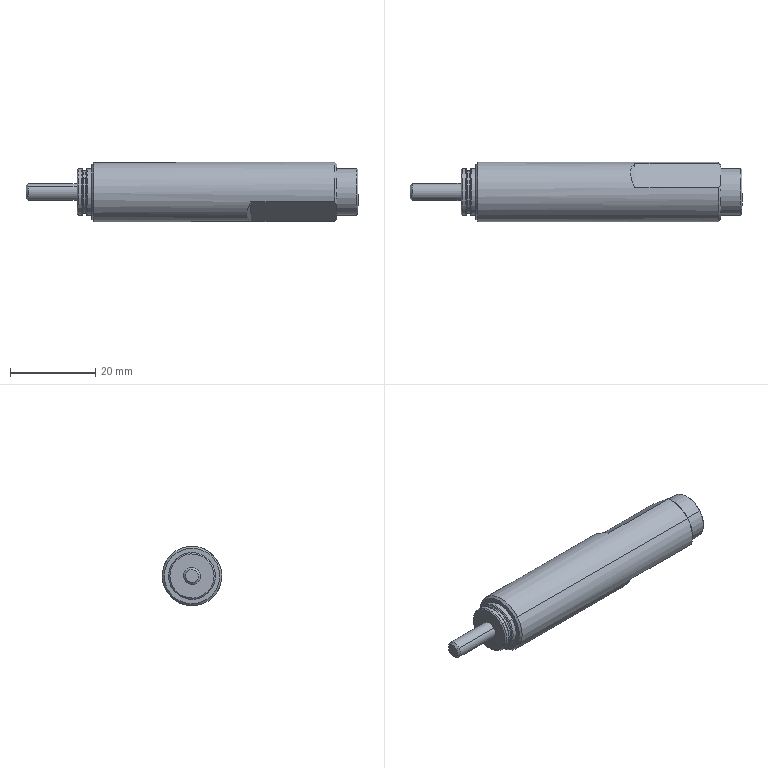Component | SolidWorks | BufferAIRTACACA_1412_2_N-1_ACA_1412_2_N_Body-1 | 1 solid | 56 faces | box 78 x 14 x 14 mm | volume 9572 mm3 | plane 19 | cone 15 | cylinder 14 | torus 8 | commonest cylinder face diameters 11 x6 2.459 x2 14 x2 10 x2 4 x2
build123d program:
from build123d import *

# Parameters (mm, degrees)
EXTRUDE1_DEPTH      = 2.5
EXTRUDE2_DEPTH      = 14
EXTRUDE2_DEPTH_BACK = 14


with BuildPart() as part:
    # Sketch1 → Revolve1 (revolve)
    with BuildSketch(Plane.XY, mode=Mode.PRIVATE) as revolve1_sk:
        with BuildLine():
            Line((0, 78), (1.5, 78))
            Line((1.5, 78), (2, 77.5))
            Line((2, 77.5), (2, 66))
            Line((2, 66), (5.2, 66))
            Line((5.2, 66), (5.5, 65.7))
            Line((5.5, 65.7), (5.5, 64.95))
            ThreePointArc((5.5, 64.95), (5.441, 64.809), (5.3, 64.75))
            Line((5.3, 64.75), (5.2, 64.75))
            ThreePointArc((5.2, 64.75), (5.059, 64.691), (5, 64.55))
            Line((5, 64.55), (5, 63.95))
            ThreePointArc((5, 63.95), (5.059, 63.809), (5.2, 63.75))
            Line((5.2, 63.75), (5.3, 63.75))
            ThreePointArc((5.3, 63.75), (5.441, 63.691), (5.5, 63.55))
            Line((5.5, 63.55), (5.5, 62.5))
            Line((5.5, 62.5), (6.54, 62.5))
            Line((6.54, 62.5), (7, 62.04))
            Line((7, 62.04), (7, 5.46))
            Line((7, 5.46), (6.54, 5))
            Line((6.54, 5), (5.5, 5))
            Line((5.5, 5), (5.5, 0.3))
            Line((5.5, 0.3), (5.2, 0))
            Line((5.2, 0), (0, 0))
            Line((0, 0), (0, 78))
        make_face()
    revolve(revolve1_sk.sketch.rotate(Axis((0, 0, 0), (0, 1, 0)), 270), axis=Axis((0, 0, 0), (0, 1, 0)))

    # Sketch2 → Cut-Revolve1 (revolve, cut)
    with BuildSketch(Plane.XY, mode=Mode.PRIVATE) as cut_revolve1_sk:
        Polygon((0, 1.2), (1.5, 1.2), (1.23, 0.9295), (1.23, 0.2705), (1.5, 0), (0, 0), align=None)
    revolve(cut_revolve1_sk.sketch.rotate(Axis((0, 0, 0), (0, 1, 0)), 180), axis=Axis((0, 0, 0), (0, 1, 0)), mode=Mode.SUBTRACT)

    # Sketch3 → Extrude1 (cut)
    with BuildSketch(Plane(origin=(0, 0, 0), x_dir=(1, 0, 0), z_dir=(0, 1, 0))):
        Polygon((-0.6495, -0.375), (0, -0.75), (0.6495, -0.375), (0.6495, 0.375), (0, 0.75), (-0.6495, 0.375), align=None)
    extrude(amount=EXTRUDE1_DEPTH, mode=Mode.SUBTRACT)

    # Sketch4 → Extrude2 (cut, two sides: drawn at the far end of the back side and taken through both)
    with BuildSketch(Plane.XY.offset(-EXTRUDE2_DEPTH_BACK)):
        Polygon((-7, -1), (7, -1), (7, 26.177), (6, 25.177), (6, 0), (-6, 0), (-6, 25.177), (-7, 26.177), align=None)
    extrude(amount=EXTRUDE2_DEPTH + EXTRUDE2_DEPTH_BACK, mode=Mode.SUBTRACT)


solid = part.part

# Placed as in the assembly
solid = solid.moved(Location((116.5, -18.6, -55), (-129.519, 0, 90)))